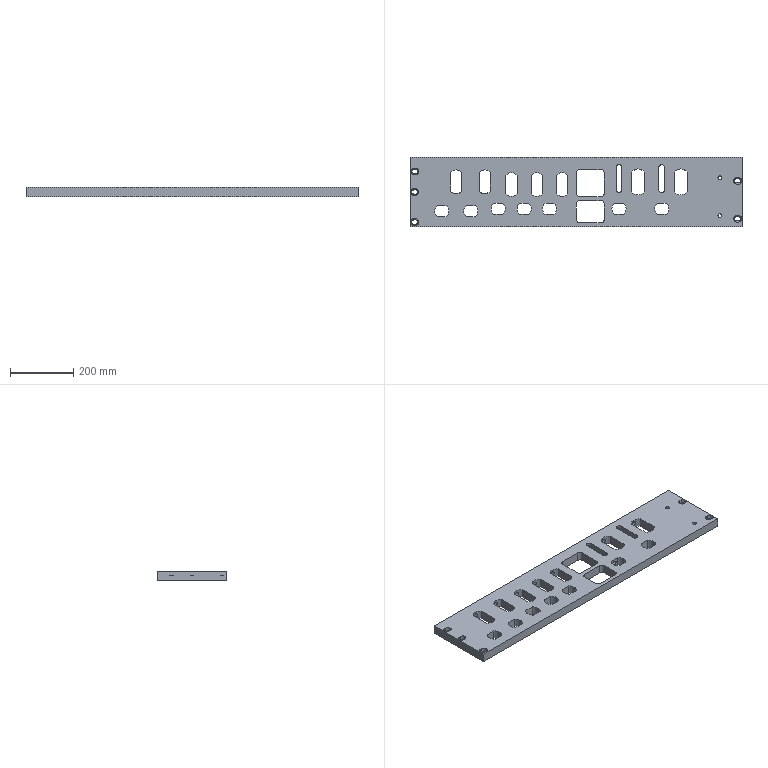Component | SolidWorks | 12AStraighteningPlate-1 | 1 solid | 192 faces | box 1050 x 220 x 28.5 mm | volume 5170872 mm3 | cylinder 111 | plane 71 | cone 10 | commonest cylinder face diameters 45 x31 20 x23 14 x22 13 x15 15.5 x8 12 x4 52 x4 18 x4 | material Q235
build123d program:
from build123d import *

# Parameters (mm, degrees)
SKETCH1_W               = 1050
SKETCH1_H               = 220
BOSS_EXTRUDE1_DEPTH     = 28.5
CUT_EXTRUDE1_DEPTH      = 28.5
HOLE1_D                 = 13
HOLE1_DEPTH             = 28.5
HOLE1_CBORE_D           = 20
HOLE1_CBORE_DEPTH       = 13
HOLE1_TIP               = 3.906
HOLE2_D                 = 13
HOLE2_DEPTH             = 28.5
HOLE2_CBORE_D           = 20
HOLE2_CBORE_DEPTH       = 13
HOLE2_TIP               = 3.906
M16_TAPPED_HOLE1_D      = 14
M16_TAPPED_HOLE1_DEPTH  = 140
M16_TAPPED_HOLE1_TIP    = 4.206
M16_TAPPED_HOLE2_REACH  = 1075.179
M16_TAPPED_HOLE2_BORE_R = 7
CUT_EXTRUDE3_DEPTH      = 13
CUT_EXTRUDE4_DEPTH      = 1073.912
SKETCH18_R              = 6
CUT_EXTRUDE5_DEPTH      = 1074.179
M18_TAPPED_HOLE1_D      = 15.5
M18_TAPPED_HOLE1_DEPTH  = 44.5
M18_TAPPED_HOLE1_TIP    = 4.657
CUT_EXTRUDE6_DEPTH      = 260


with BuildPart() as part:
    # Sketch1 → Boss-Extrude1 (new body)
    with BuildSketch(Plane.XY):
        with Locations((525, -110)):
            Rectangle(SKETCH1_W, SKETCH1_H)
    extrude(amount=BOSS_EXTRUDE1_DEPTH)

    # Sketch2 → Cut-Extrude1 (cut)
    with BuildSketch(Plane.XY.offset(28.5)):
        with BuildLine():
            Line((128.5, -48.358), (128.5, -107.642))
            ThreePointArc((128.5, -107.642), (146, -116), (163.5, -107.642))
            Line((163.5, -107.642), (163.5, -48.358))
            ThreePointArc((163.5, -48.358), (146, -40), (128.5, -48.358))
        make_face()
        with BuildLine():
            Line((218.5, -48.358), (218.5, -107.642))
            ThreePointArc((218.5, -107.642), (236, -116), (253.5, -107.642))
            Line((253.5, -107.642), (253.5, -48.358))
            ThreePointArc((253.5, -48.358), (236, -40), (218.5, -48.358))
        make_face()
        with BuildLine():
            Line((338.5, -56.858), (338.5, -116.142))
            ThreePointArc((338.5, -116.142), (321, -124.5), (303.5, -116.142))
            Line((303.5, -116.142), (303.5, -56.858))
            ThreePointArc((303.5, -56.858), (321, -48.5), (338.5, -56.858))
        make_face()
        with BuildLine():
            Line((383.5, -56.858), (383.5, -116.142))
            ThreePointArc((383.5, -116.142), (401, -124.5), (418.5, -116.142))
            Line((418.5, -116.142), (418.5, -56.858))
            ThreePointArc((418.5, -56.858), (401, -48.5), (383.5, -56.858))
        make_face()
        with BuildLine():
            Line((498.5, -56.858), (498.5, -116.142))
            ThreePointArc((498.5, -116.142), (481, -124.5), (463.5, -116.142))
            Line((463.5, -116.142), (463.5, -56.858))
            ThreePointArc((463.5, -56.858), (481, -48.5), (498.5, -56.858))
        make_face()
        with BuildLine():
            Line((85.858, -153.5), (114.142, -153.5))
            ThreePointArc((114.142, -153.5), (122.5, -171), (114.142, -188.5))
            Line((114.142, -188.5), (85.858, -188.5))
            ThreePointArc((85.858, -188.5), (77.5, -171), (85.858, -153.5))
        make_face()
        with BuildLine():
            Line((177.858, -153.5), (206.142, -153.5))
            ThreePointArc((206.142, -153.5), (214.5, -171), (206.142, -188.5))
            Line((206.142, -188.5), (177.858, -188.5))
            ThreePointArc((177.858, -188.5), (169.5, -171), (177.858, -153.5))
        make_face()
        with BuildLine():
            Line((426.858, -181), (455.142, -181))
            ThreePointArc((455.142, -181), (463.5, -163.5), (455.142, -146))
            Line((455.142, -146), (426.858, -146))
            ThreePointArc((426.858, -146), (418.5, -163.5), (426.858, -181))
        make_face()
        with BuildLine():
            Line((264.858, -181), (293.142, -181))
            ThreePointArc((293.142, -181), (301.5, -163.5), (293.142, -146))
            Line((293.142, -146), (264.858, -146))
            ThreePointArc((264.858, -146), (256.5, -163.5), (264.858, -181))
        make_face()
        with BuildLine():
            Line((346.858, -181), (375.142, -181))
            ThreePointArc((375.142, -181), (383.5, -163.5), (375.142, -146))
            Line((375.142, -146), (346.858, -146))
            ThreePointArc((346.858, -146), (338.5, -163.5), (346.858, -181))
        make_face()
        with BuildLine():
            Line((646.858, -146), (675.142, -146))
            ThreePointArc((675.142, -146), (683.5, -163.5), (675.142, -181))
            Line((675.142, -181), (646.858, -181))
            ThreePointArc((646.858, -181), (638.5, -163.5), (646.858, -146))
        make_face()
        with BuildLine():
            Line((781.858, -181), (810.142, -181))
            ThreePointArc((810.142, -181), (818.5, -163.5), (810.142, -146))
            Line((810.142, -146), (781.858, -146))
            ThreePointArc((781.858, -146), (773.5, -163.5), (781.858, -181))
        make_face()
        with BuildLine():
            Line((700.5, -47.008), (700.5, -108.992))
            ThreePointArc((700.5, -108.992), (721, -119), (741.5, -108.992))
            Line((741.5, -108.992), (741.5, -47.008))
            ThreePointArc((741.5, -47.008), (721, -37), (700.5, -47.008))
        make_face()
        with BuildLine():
            Line((876.5, -47.008), (876.5, -108.992))
            ThreePointArc((876.5, -108.992), (856, -119), (835.5, -108.992))
            Line((835.5, -108.992), (835.5, -47.008))
            ThreePointArc((835.5, -47.008), (856, -37), (876.5, -47.008))
        make_face()
        with BuildLine():
            Line((670, -32.5), (670, -103.5))
            ThreePointArc((670, -103.5), (661, -112.5), (652, -103.5))
            Line((652, -103.5), (652, -32.5))
            ThreePointArc((652, -32.5), (661, -23.5), (670, -32.5))
        make_face()
        with BuildLine():
            Line((787, -32.5), (787, -103.5))
            ThreePointArc((787, -103.5), (796, -112.5), (805, -103.5))
            Line((805, -103.5), (805, -32.5))
            ThreePointArc((805, -32.5), (796, -23.5), (787, -32.5))
        make_face()
    extrude(amount=-CUT_EXTRUDE1_DEPTH, mode=Mode.SUBTRACT)

    # Hole1
    with Locations(Plane.XY.offset(28.5)):
        with Locations((1036.5, -75), (1036.5, -195)):
            CounterBoreHole(HOLE1_D / 2, HOLE1_CBORE_D / 2, HOLE1_CBORE_DEPTH, depth=HOLE1_DEPTH)
            with Locations((0, 0, -(HOLE1_DEPTH + HOLE1_TIP / 2))):  # 118° drill point
                Cone(0, HOLE1_D / 2, HOLE1_TIP, mode=Mode.SUBTRACT)

    # Hole2
    with Locations(Plane.XY.offset(28.5)):
        with Locations((15, -205), (15, -110), (15, -45)):
            CounterBoreHole(HOLE2_D / 2, HOLE2_CBORE_D / 2, HOLE2_CBORE_DEPTH, depth=HOLE2_DEPTH)
            with Locations((0, 0, -(HOLE2_DEPTH + HOLE2_TIP / 2))):  # 118° drill point
                Cone(0, HOLE2_D / 2, HOLE2_TIP, mode=Mode.SUBTRACT)

    # M16 Tapped Hole1
    with Locations(Plane(origin=(0, 0, 0), x_dir=(1, 0, 0), z_dir=(0, 1, 0))):
        with Locations((661, -14.25), (146, -14.25), (236, -14.25), (321, -14.25), (401, -14.25), (481, -14.25)):
            Hole(M16_TAPPED_HOLE1_D / 2, depth=M16_TAPPED_HOLE1_DEPTH)
            with Locations((0, 0, -(M16_TAPPED_HOLE1_DEPTH + M16_TAPPED_HOLE1_TIP / 2))):  # 118° drill point
                Cone(0, M16_TAPPED_HOLE1_D / 2, M16_TAPPED_HOLE1_TIP, mode=Mode.SUBTRACT)

    # M16 Tapped Hole2 bore → M16 Tapped Hole2 (cut, up to next)
    with BuildSketch(Plane(origin=(0, 0, 0), x_dir=(1, 0, 0), z_dir=(0, 1, 0)), mode=Mode.PRIVATE) as m16_tapped_hole2_sk1:
        with Locations((856, -14.25)):
            Circle(M16_TAPPED_HOLE2_BORE_R)
    m16_tapped_hole2_tool1 = extrude(m16_tapped_hole2_sk1.sketch, amount=-M16_TAPPED_HOLE2_REACH, mode=Mode.PRIVATE) & part.part
    # M16 Tapped Hole2 bore → M16 Tapped Hole2 (cut, up to next)
    with BuildSketch(Plane(origin=(0, 0, 0), x_dir=(1, 0, 0), z_dir=(0, 1, 0)), mode=Mode.PRIVATE) as m16_tapped_hole2_sk2:
        with Locations((661, -14.25)):
            Circle(M16_TAPPED_HOLE2_BORE_R)
    m16_tapped_hole2_tool2 = extrude(m16_tapped_hole2_sk2.sketch, amount=-M16_TAPPED_HOLE2_REACH, mode=Mode.PRIVATE) & part.part
    # M16 Tapped Hole2 bore → M16 Tapped Hole2 (cut, up to next)
    with BuildSketch(Plane(origin=(0, 0, 0), x_dir=(1, 0, 0), z_dir=(0, 1, 0)), mode=Mode.PRIVATE) as m16_tapped_hole2_sk3:
        with Locations((796, -14.25)):
            Circle(M16_TAPPED_HOLE2_BORE_R)
    m16_tapped_hole2_tool3 = extrude(m16_tapped_hole2_sk3.sketch, amount=-M16_TAPPED_HOLE2_REACH, mode=Mode.PRIVATE) & part.part
    # M16 Tapped Hole2 bore → M16 Tapped Hole2 (cut, up to next)
    with BuildSketch(Plane(origin=(0, 0, 0), x_dir=(1, 0, 0), z_dir=(0, 1, 0)), mode=Mode.PRIVATE) as m16_tapped_hole2_sk4:
        with Locations((721, -14.25)):
            Circle(M16_TAPPED_HOLE2_BORE_R)
    m16_tapped_hole2_tool4 = extrude(m16_tapped_hole2_sk4.sketch, amount=-M16_TAPPED_HOLE2_REACH, mode=Mode.PRIVATE) & part.part
    add(m16_tapped_hole2_tool1.solids().sort_by_distance((856, 0, 14.25))[0], mode=Mode.SUBTRACT)
    add(m16_tapped_hole2_tool2.solids().sort_by_distance((661, 0, 14.25))[0], mode=Mode.SUBTRACT)
    add(m16_tapped_hole2_tool3.solids().sort_by_distance((796, 0, 14.25))[0], mode=Mode.SUBTRACT)
    add(m16_tapped_hole2_tool4.solids().sort_by_distance((721, 0, 14.25))[0], mode=Mode.SUBTRACT)

    # Sketch16 → Cut-Extrude3 (cut)
    with BuildSketch(Plane.XY.offset(28.5)):
        with BuildLine():
            Line((1033.25, -65), (1039.75, -65))
            ThreePointArc((1039.75, -65), (1049.75, -75), (1039.75, -85))
            Line((1039.75, -85), (1033.25, -85))
            ThreePointArc((1033.25, -85), (1023.25, -75), (1033.25, -65))
        make_face()
        with BuildLine():
            Line((11.75, -35), (18.25, -35))
            ThreePointArc((18.25, -35), (28.25, -45), (18.25, -55))
            Line((18.25, -55), (11.75, -55))
            ThreePointArc((11.75, -55), (1.75, -45), (11.75, -35))
        make_face()
        with BuildLine():
            Line((1033.25, -185), (1039.75, -185))
            ThreePointArc((1039.75, -185), (1049.75, -195), (1039.75, -205))
            Line((1039.75, -205), (1033.25, -205))
            ThreePointArc((1033.25, -205), (1023.25, -195), (1033.25, -185))
        make_face()
        with BuildLine():
            Line((11.75, -100), (18.25, -100))
            ThreePointArc((18.25, -100), (28.25, -110), (18.25, -120))
            Line((18.25, -120), (11.75, -120))
            ThreePointArc((11.75, -120), (1.75, -110), (11.75, -100))
        make_face()
        with BuildLine():
            Line((11.75, -195), (18.25, -195))
            ThreePointArc((18.25, -195), (28.25, -205), (18.25, -215))
            Line((18.25, -215), (11.75, -215))
            ThreePointArc((11.75, -215), (1.75, -205), (11.75, -195))
        make_face()
    extrude(amount=-CUT_EXTRUDE3_DEPTH, mode=Mode.SUBTRACT)

    # Sketch17 → Cut-Extrude4 (cut, through all)
    with BuildSketch(Plane.XY.offset(15.5)):
        with BuildLine():
            Line((1033.25, -68.5), (1039.75, -68.5))
            ThreePointArc((1039.75, -68.5), (1046.25, -75), (1039.75, -81.5))
            Line((1039.75, -81.5), (1033.25, -81.5))
            ThreePointArc((1033.25, -81.5), (1026.75, -75), (1033.25, -68.5))
        make_face()
        with BuildLine():
            Line((11.75, -38.5), (18.25, -38.5))
            ThreePointArc((18.25, -38.5), (24.75, -45), (18.25, -51.5))
            Line((18.25, -51.5), (11.75, -51.5))
            ThreePointArc((11.75, -51.5), (5.25, -45), (11.75, -38.5))
        make_face()
        with BuildLine():
            Line((1033.25, -188.5), (1039.75, -188.5))
            ThreePointArc((1039.75, -188.5), (1046.25, -195), (1039.75, -201.5))
            Line((1039.75, -201.5), (1033.25, -201.5))
            ThreePointArc((1033.25, -201.5), (1026.75, -195), (1033.25, -188.5))
        make_face()
        with BuildLine():
            Line((11.75, -103.5), (18.25, -103.5))
            ThreePointArc((18.25, -103.5), (24.75, -110), (18.25, -116.5))
            Line((18.25, -116.5), (11.75, -116.5))
            ThreePointArc((11.75, -116.5), (5.25, -110), (11.75, -103.5))
        make_face()
        with BuildLine():
            Line((11.75, -198.5), (18.25, -198.5))
            ThreePointArc((18.25, -198.5), (24.75, -205), (18.25, -211.5))
            Line((18.25, -211.5), (11.75, -211.5))
            ThreePointArc((11.75, -211.5), (5.25, -205), (11.75, -198.5))
        make_face()
    extrude(amount=-CUT_EXTRUDE4_DEPTH, mode=Mode.SUBTRACT)

    # Sketch18 → Cut-Extrude5 (cut, through all)
    with BuildSketch(Plane.XY.offset(28.5)):
        with Locations((980, -185)):
            Circle(SKETCH18_R)
        with Locations((980, -65)):
            Circle(SKETCH18_R)
    extrude(amount=-CUT_EXTRUDE5_DEPTH, mode=Mode.SUBTRACT)

    # M18 Tapped Hole1
    with Locations(Plane(origin=(0, 0, 0), x_dir=(1, 0, 0), z_dir=(0, 1, 0))):
        with Locations((661, -14.25), (721, -14.25), (796, -14.25), (856, -14.25)):
            Hole(M18_TAPPED_HOLE1_D / 2, depth=M18_TAPPED_HOLE1_DEPTH)
            with Locations((0, 0, -(M18_TAPPED_HOLE1_DEPTH + M18_TAPPED_HOLE1_TIP / 2))):  # 118° drill point
                Cone(0, M18_TAPPED_HOLE1_D / 2, M18_TAPPED_HOLE1_TIP, mode=Mode.SUBTRACT)

    # Sketch25 → Cut-Extrude6 (cut)
    with BuildSketch(Plane.XY.offset(28.5)):
        with BuildLine():
            Line((536.295, -137.367), (604.295, -137.367))
            ThreePointArc((604.295, -137.367), (611.366, -140.296), (614.295, -147.367))
            Line((614.295, -147.367), (614.295, -197.367))
            ThreePointArc((614.295, -197.367), (611.366, -204.438), (604.295, -207.367))
            Line((604.295, -207.367), (536.295, -207.367))
            ThreePointArc((536.295, -207.367), (529.224, -204.438), (526.295, -197.367))
            Line((526.295, -197.367), (526.295, -147.367))
            ThreePointArc((526.295, -147.367), (529.224, -140.296), (536.295, -137.367))
        make_face()
        with BuildLine():
            Line((536.295, -39.367), (604.295, -39.367))
            ThreePointArc((604.295, -39.367), (611.366, -42.296), (614.295, -49.367))
            Line((614.295, -49.367), (614.295, -114.367))
            ThreePointArc((614.295, -114.367), (611.366, -121.438), (604.295, -124.367))
            Line((604.295, -124.367), (536.295, -124.367))
            ThreePointArc((536.295, -124.367), (529.224, -121.438), (526.295, -114.367))
            Line((526.295, -114.367), (526.295, -49.367))
            ThreePointArc((526.295, -49.367), (529.224, -42.296), (536.295, -39.367))
        make_face()
    extrude(amount=-CUT_EXTRUDE6_DEPTH, mode=Mode.SUBTRACT)


solid = part.part

# Placed as in the assembly
solid = solid.moved(Location((-449.402, 230.038, -14.25), (0, 0, 0)))